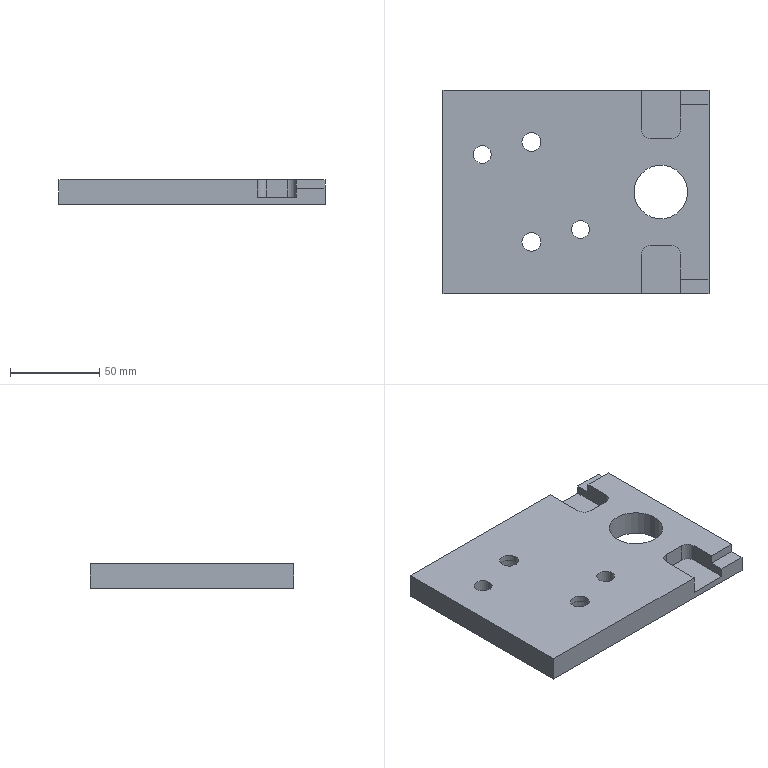Component | NX | BASE_PLATE | 1 solid | 31 faces | volume 208195 mm3 | plane 20 | cylinder 11 | commonest cylinder face diameters 10 x6 10.5 x2 15.5 x2 30 x1